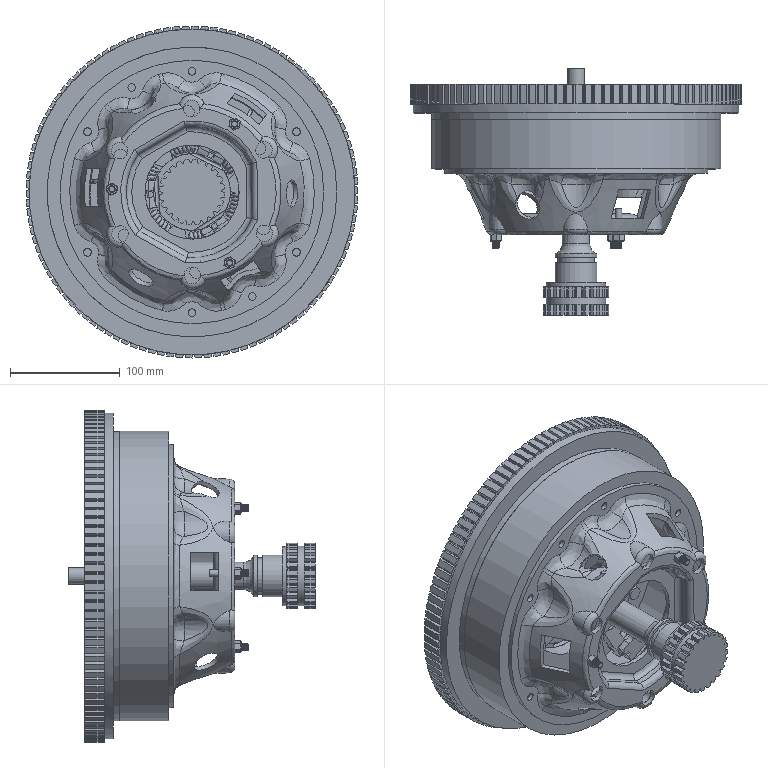Assembly | NX | mm | 16 component files | 16 solids | 1536 faces | box 302.66 x 225 x 302.67 mm | volume 3697041 mm3 | plane 992 | cylinder 336 | spline 113 | cone 68 | torus 27 | commonest cylinder face diameters 60 x48 6 x22 25 x22 7 x20 12 x18 6.8 x18 10.114 x16 30 x13
Bill of materials:
unnamed part 1 | 3 |  | Stepped cylindrical pin with three coaxial sections: an externally threaded end, a larger-diameter plain collar, and a smaller plain cylindrical shank at the other end.
unnamed part 2 | 1 |  | Flat annular disc with a central round hole and small raised tabs or stepped blocks on one face. The outer rim has flat chord cuts and small edge notches.
unnamed part 3 | 3 |  | Elongated hexagonal body with a plain cylindrical through-bore along its axis and chamfered ends. It is about twice as long as it is across the flats.
unnamed part 4 | 1 |  | Thin circular disc with a central hub that has an internally splined/toothed bore. Six helical coil springs sit in windows arranged around the hub. The outer annulus has a ring of small holes and arc-shaped slots.
unnamed part 5 | 1 |  | Large flat circular disc with many fine teeth around its outer periphery. It has a central round bore, a small inner hole pattern and an outer hole pattern, and stepped raised/recessed faces on one side.
unnamed part 6 | 1 |  | Flat annular ring with blocky multi-step tab/clip features on one face at two or three locations. The face has small holes and a radial split or cut in the ring.
unnamed part 7 | 3 |  | Small bent-plate bracket or lever with a rectangular window and a forked slotted end. It has a transverse cylindrical pivot bore through side lugs near one end, plus curved hooked flanges.
unnamed part 8 | 1 |  | Dished, cup-shaped shell with a flat outer flange ringed by small holes and a conical/tapered wall with round and quadrilateral openings. The base is a flat annular face with a central round bore and larger bolt holes, inside a polygonal recess.
unnamed part 9 | 1 |  | Plain rectangular-section ring (short thick-walled tube) with a pattern of small axial holes in one end face.
unnamed part 10 | 1 |  | Stepped shaft with a toothed/splined head at one end made of two axially separated tooth bands, a neck groove and fillet, and a long plain shank. The shank carries a spline or keyway section and a smaller-diameter pilot end.
Mates:
1. fix | Clutch_Cover 1 component
2. touch align | Clutch_Cover 1 face | Drive_Shaft_Flywheel 1 face
3. concentric | Spring_Pressure_Friction_Plate 1 edge | Drive_Shaft_Flywheel 1 edge
4. touch align | Clutch_Pressure_Plate 1 face | Spring_Pressure_Friction_Plate 1 face
5. touch align | Spring_Pressure_Friction_Plate 1 face | Clutch_Pressure_Plate 1 face
6. center | Lever 3 face | Lever 3 face | Clutch_Pressure_Plate 1 face | Clutch_Pressure_Plate 1 face
7. touch align | Lever 3 face | Clutch_Pressure_Plate 1 face
8. bond | Spring_Pressure_Friction_Plate 1 component | assembly component
9. bond | Lever 3 component | assembly component
10. bond | Lever 2 component | assembly component
11. bond | Lever 1 component | assembly component
12. circular | assembly datumaxis | assembly cartesiancoordinatesystem | assembly cartesiancoordinatesystem | assembly cartesiancoordinatesystem
13. touch align | Drive_Flange 1 face | Clutch_Pressure_Plate 1 face
14. touch align | Drive_Flange 1 face | Lever 3 face
15. parallel | Drive_Flange 1 face | Lever 3 face
16. touch align | Drive_Shaft 1 face | Drive_Flange 1 face
17. parallel | Drive_Shaft 1 face | Spring_Pressure_Friction_Plate 1 face
18. touch align | Clutch_Pressure_Plate 1 face | Clutch_Cover 1 face
19. touch align | Clutch_Cover 1 face | Drive_Shaft_Flywheel 1 face
20. touch align | Drive_Shaft 1 face | Spring_Pressure_Friction_Plate 1 face
21. concentric | Intermediate_Connector 1 edge | Drive_Shaft_Flywheel 1 edge
22. touch align | Intermediate_Connector 1 face | Clutch_Pressure_Plate 1 face
23. concentric | Stud 3 edge | Clutch_Cover 1 edge
24. bond | Drive_Shaft 1 component | assembly component
25. bond | Stud 3 component | assembly component
26. bond | Stud 2 component | assembly component
27. bond | Stud 1 component | assembly component
28. circular | assembly datumaxis | assembly cartesiancoordinatesystem | assembly cartesiancoordinatesystem | assembly cartesiancoordinatesystem
29. concentric | Hex_Lock_Nut_M6_GB_T_6184 3 edge | Clutch_Cover 1 edge
30. bond | Drive_Shaft 1 component | assembly component
31. bond | Hex_Lock_Nut_M6_GB_T_6184 3 component | assembly component
32. bond | Hex_Lock_Nut_M6_GB_T_6184 2 component | assembly component
33. bond | Hex_Lock_Nut_M6_GB_T_6184 1 component | assembly component
34. circular | assembly datumaxis | assembly cartesiancoordinatesystem | assembly cartesiancoordinatesystem | assembly cartesiancoordinatesystem